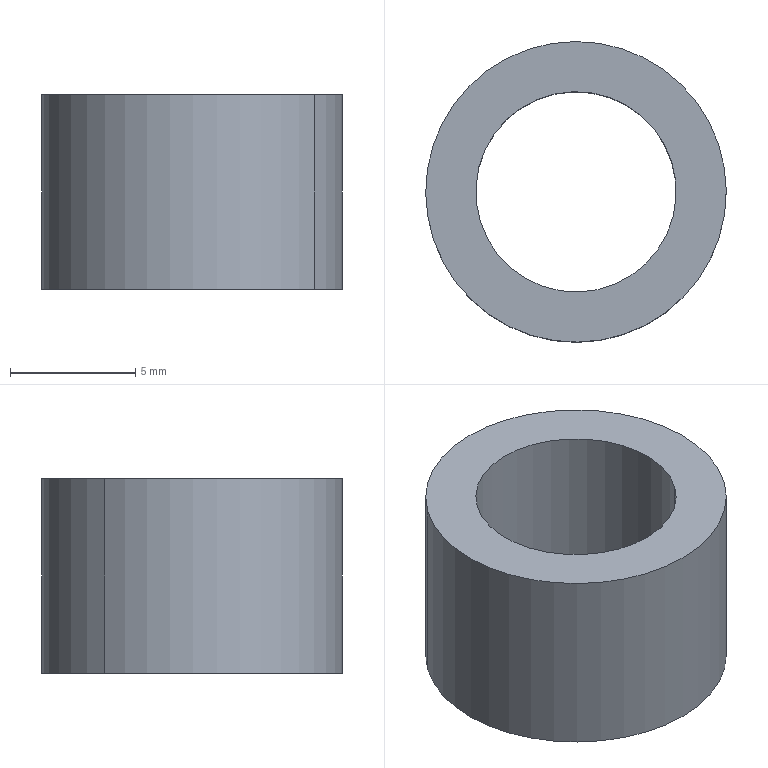Component | SolidWorks | 10BoltSleeve-Length7.75-2 | 1 solid | 6 faces | box 12 x 12 x 7.75 mm | volume 487 mm3 | cylinder 4 | plane 2 | commonest cylinder face diameters 8 x2 12 x2
build123d program:
from build123d import *

# Parameters (mm, degrees)
SKETCH1_R           = 6
SKETCH1_R_2         = 4
BOSS_EXTRUDE1_DEPTH = 7.75


with BuildPart() as part:
    # Sketch1 → Boss-Extrude1 (new body)
    with BuildSketch(Plane.XY):
        Circle(SKETCH1_R)
        Circle(SKETCH1_R_2, mode=Mode.SUBTRACT)
    extrude(amount=BOSS_EXTRUDE1_DEPTH)


solid = part.part

# Placed as in the assembly
solid = solid.moved(Location((94.618, 134.462, 31.788), (0, 0, 0)))
STEP:
#1=COLOUR_RGB('',0.7922,0.8196,0.9333);
#2=FILL_AREA_STYLE_COLOUR('',#1);
#3=FILL_AREA_STYLE('',(#2));
#4=SURFACE_STYLE_FILL_AREA(#3);
#5=SURFACE_SIDE_STYLE('',(#4));
#6=SURFACE_STYLE_USAGE(.BOTH.,#5);
#7=PRESENTATION_STYLE_ASSIGNMENT((#6));
#8=CARTESIAN_POINT('',(3.597,5.385,1.557));
#9=VERTEX_POINT('',#8);
#10=CARTESIAN_POINT('',(3.853,5.202,1.557));
#11=VERTEX_POINT('',#10);
#12=CARTESIAN_POINT('',(3.725,5.294,1.557));
#13=DIRECTION('',(0.,0.,1.));
#14=DIRECTION('',(0.8135,-0.5816,0.));
#15=AXIS2_PLACEMENT_3D('',#12,#13,#14);
#16=CIRCLE('',#15,0.1575);
#17=EDGE_CURVE('',#9,#11,#16,.T.);
#18=ORIENTED_EDGE('',*,*,#17,.T.);
#19=CARTESIAN_POINT('',(3.853,5.202,1.251));
#20=VERTEX_POINT('',#19);
#21=CARTESIAN_POINT('',(3.853,5.202,1.557));
#22=DIRECTION('',(0.,0.,-1.));
#23=VECTOR('',#22,39.37);
#24=LINE('',#21,#23);
#25=EDGE_CURVE('',#11,#20,#24,.T.);
#26=ORIENTED_EDGE('',*,*,#25,.T.);
#27=CARTESIAN_POINT('',(3.597,5.385,1.251));
#28=VERTEX_POINT('',#27);
#29=CARTESIAN_POINT('',(3.725,5.294,1.251));
#30=DIRECTION('',(0.,0.,1.));
#31=DIRECTION('',(0.8135,-0.5816,0.));
#32=AXIS2_PLACEMENT_3D('',#29,#30,#31);
#33=CIRCLE('',#32,0.1575);
#34=EDGE_CURVE('',#28,#20,#33,.T.);
#35=ORIENTED_EDGE('',*,*,#34,.F.);
#36=CARTESIAN_POINT('',(3.597,5.385,1.557));
#37=DIRECTION('',(0.,0.,-1.));
#38=VECTOR('',#37,39.37);
#39=LINE('',#36,#38);
#40=EDGE_CURVE('',#9,#28,#39,.T.);
#41=ORIENTED_EDGE('',*,*,#40,.F.);
#42=EDGE_LOOP('',(#18,#26,#35,#41));
#43=FACE_OUTER_BOUND('',#42,.T.);
#44=CARTESIAN_POINT('',(3.725,5.294,1.557));
#45=DIRECTION('',(0.,0.,-1.));
#46=DIRECTION('',(-0.8135,0.5816,0.));
#47=AXIS2_PLACEMENT_3D('',#44,#45,#46);
#48=CYLINDRICAL_SURFACE('',#47,0.1575);
#49=ADVANCED_FACE('',(#43),#48,.F.);
#50=CARTESIAN_POINT('',(3.917,5.156,1.557));
#51=VERTEX_POINT('',#50);
#52=CARTESIAN_POINT('',(3.533,5.431,1.557));
#53=VERTEX_POINT('',#52);
#54=CARTESIAN_POINT('',(3.725,5.294,1.557));
#55=DIRECTION('',(0.,0.,1.));
#56=DIRECTION('',(0.8135,-0.5816,0.));
#57=AXIS2_PLACEMENT_3D('',#54,#55,#56);
#58=CIRCLE('',#57,0.2362);
#59=EDGE_CURVE('',#51,#53,#58,.T.);
#60=ORIENTED_EDGE('',*,*,#59,.F.);
#61=CARTESIAN_POINT('',(3.917,5.156,1.251));
#62=VERTEX_POINT('',#61);
#63=CARTESIAN_POINT('',(3.917,5.156,1.557));
#64=DIRECTION('',(0.,0.,-1.));
#65=VECTOR('',#64,39.37);
#66=LINE('',#63,#65);
#67=EDGE_CURVE('',#51,#62,#66,.T.);
#68=ORIENTED_EDGE('',*,*,#67,.T.);
#69=CARTESIAN_POINT('',(3.533,5.431,1.251));
#70=VERTEX_POINT('',#69);
#71=CARTESIAN_POINT('',(3.725,5.294,1.251));
#72=DIRECTION('',(0.,0.,1.));
#73=DIRECTION('',(0.8135,-0.5816,0.));
#74=AXIS2_PLACEMENT_3D('',#71,#72,#73);
#75=CIRCLE('',#74,0.2362);
#76=EDGE_CURVE('',#62,#70,#75,.T.);
#77=ORIENTED_EDGE('',*,*,#76,.T.);
#78=CARTESIAN_POINT('',(3.533,5.431,1.557));
#79=DIRECTION('',(0.,0.,-1.));
#80=VECTOR('',#79,39.37);
#81=LINE('',#78,#80);
#82=EDGE_CURVE('',#53,#70,#81,.T.);
#83=ORIENTED_EDGE('',*,*,#82,.F.);
#84=EDGE_LOOP('',(#60,#68,#77,#83));
#85=FACE_OUTER_BOUND('',#84,.T.);
#86=CARTESIAN_POINT('',(3.725,5.294,1.557));
#87=DIRECTION('',(0.,0.,-1.));
#88=DIRECTION('',(-0.8135,0.5816,0.));
#89=AXIS2_PLACEMENT_3D('',#86,#87,#88);
#90=CYLINDRICAL_SURFACE('',#89,0.2362);
#91=ADVANCED_FACE('',(#85),#90,.T.);
#92=CARTESIAN_POINT('',(3.725,5.294,1.557));
#93=DIRECTION('',(0.,0.,1.));
#94=DIRECTION('',(0.8135,-0.5816,0.));
#95=AXIS2_PLACEMENT_3D('',#92,#93,#94);
#96=CIRCLE('',#95,0.2362);
#97=EDGE_CURVE('',#53,#51,#96,.T.);
#98=ORIENTED_EDGE('',*,*,#97,.T.);
#99=ORIENTED_EDGE('',*,*,#59,.T.);
#100=EDGE_LOOP('',(#98,#99));
#101=FACE_OUTER_BOUND('',#100,.T.);
#102=ORIENTED_EDGE('',*,*,#17,.F.);
#103=CARTESIAN_POINT('',(3.725,5.294,1.557));
#104=DIRECTION('',(0.,0.,1.));
#105=DIRECTION('',(0.8135,-0.5816,0.));
#106=AXIS2_PLACEMENT_3D('',#103,#104,#105);
#107=CIRCLE('',#106,0.1575);
#108=EDGE_CURVE('',#11,#9,#107,.T.);
#109=ORIENTED_EDGE('',*,*,#108,.F.);
#110=EDGE_LOOP('',(#102,#109));
#111=FACE_BOUND('',#110,.T.);
#112=CARTESIAN_POINT('',(3.725,5.294,1.557));
#113=DIRECTION('',(0.,0.,1.));
#114=DIRECTION('',(0.8135,-0.5816,0.));
#115=AXIS2_PLACEMENT_3D('',#112,#113,#114);
#116=PLANE('',#115);
#117=ADVANCED_FACE('',(#101,#111),#116,.T.);
#118=CARTESIAN_POINT('',(3.725,5.294,1.251));
#119=DIRECTION('',(0.,0.,1.));
#120=DIRECTION('',(0.8135,-0.5816,0.));
#121=AXIS2_PLACEMENT_3D('',#118,#119,#120);
#122=CIRCLE('',#121,0.2362);
#123=EDGE_CURVE('',#70,#62,#122,.T.);
#124=ORIENTED_EDGE('',*,*,#123,.F.);
#125=ORIENTED_EDGE('',*,*,#76,.F.);
#126=EDGE_LOOP('',(#124,#125));
#127=FACE_OUTER_BOUND('',#126,.T.);
#128=ORIENTED_EDGE('',*,*,#34,.T.);
#129=CARTESIAN_POINT('',(3.725,5.294,1.251));
#130=DIRECTION('',(0.,0.,1.));
#131=DIRECTION('',(0.8135,-0.5816,0.));
#132=AXIS2_PLACEMENT_3D('',#129,#130,#131);
#133=CIRCLE('',#132,0.1575);
#134=EDGE_CURVE('',#20,#28,#133,.T.);
#135=ORIENTED_EDGE('',*,*,#134,.T.);
#136=EDGE_LOOP('',(#128,#135));
#137=FACE_BOUND('',#136,.T.);
#138=CARTESIAN_POINT('',(3.725,5.294,1.251));
#139=DIRECTION('',(0.,0.,1.));
#140=DIRECTION('',(0.8135,-0.5816,0.));
#141=AXIS2_PLACEMENT_3D('',#138,#139,#140);
#142=PLANE('',#141);
#143=ADVANCED_FACE('',(#127,#137),#142,.F.);
#144=ORIENTED_EDGE('',*,*,#67,.F.);
#145=ORIENTED_EDGE('',*,*,#97,.F.);
#146=ORIENTED_EDGE('',*,*,#82,.T.);
#147=ORIENTED_EDGE('',*,*,#123,.T.);
#148=EDGE_LOOP('',(#144,#145,#146,#147));
#149=FACE_OUTER_BOUND('',#148,.T.);
#150=CARTESIAN_POINT('',(3.725,5.294,1.557));
#151=DIRECTION('',(0.,0.,-1.));
#152=DIRECTION('',(-0.8135,0.5816,0.));
#153=AXIS2_PLACEMENT_3D('',#150,#151,#152);
#154=CYLINDRICAL_SURFACE('',#153,0.2362);
#155=ADVANCED_FACE('',(#149),#154,.T.);
#156=ORIENTED_EDGE('',*,*,#25,.F.);
#157=ORIENTED_EDGE('',*,*,#108,.T.);
#158=ORIENTED_EDGE('',*,*,#40,.T.);
#159=ORIENTED_EDGE('',*,*,#134,.F.);
#160=EDGE_LOOP('',(#156,#157,#158,#159));
#161=FACE_OUTER_BOUND('',#160,.T.);
#162=CARTESIAN_POINT('',(3.725,5.294,1.557));
#163=DIRECTION('',(0.,0.,-1.));
#164=DIRECTION('',(-0.8135,0.5816,0.));
#165=AXIS2_PLACEMENT_3D('',#162,#163,#164);
#166=CYLINDRICAL_SURFACE('',#165,0.1575);
#167=ADVANCED_FACE('',(#161),#166,.F.);
#168=CLOSED_SHELL('',(#49,#91,#117,#143,#155,#167));
#169=MANIFOLD_SOLID_BREP('',#168);
#170=STYLED_ITEM('',(#7),#169);
#171=(LENGTH_UNIT()NAMED_UNIT(*)SI_UNIT($,.METRE.));
#172=LENGTH_MEASURE_WITH_UNIT(LENGTH_MEASURE(0.0254),#171);
#173=DIMENSIONAL_EXPONENTS(1.,0.,0.,0.,0.,0.,0.);
#174=(CONVERSION_BASED_UNIT('',#172)LENGTH_UNIT()NAMED_UNIT(#173));
#175=UNCERTAINTY_MEASURE_WITH_UNIT(LENGTH_MEASURE(0.00001),#174,'','');
#176=(NAMED_UNIT(*)PLANE_ANGLE_UNIT()SI_UNIT($,.RADIAN.));
#177=(NAMED_UNIT(*)SI_UNIT($,.STERADIAN.)SOLID_ANGLE_UNIT());
#178=(GEOMETRIC_REPRESENTATION_CONTEXT(3)GLOBAL_UNCERTAINTY_ASSIGNED_CONTEXT((#175))GLOBAL_UNIT_ASSIGNED_CONTEXT((#174,#176,#177))REPRESENTATION_CONTEXT('',''));
#179=MECHANICAL_DESIGN_GEOMETRIC_PRESENTATION_REPRESENTATION('',(#170),#178);
#180=CARTESIAN_POINT('',(0.,0.,0.));
#181=DIRECTION('',(0.,0.,1.));
#182=DIRECTION('',(1.,0.,0.));
#183=AXIS2_PLACEMENT_3D('',#180,#181,#182);
#184=(LENGTH_UNIT()NAMED_UNIT(*)SI_UNIT($,.METRE.));
#185=LENGTH_MEASURE_WITH_UNIT(LENGTH_MEASURE(0.0254),#184);
#186=DIMENSIONAL_EXPONENTS(1.,0.,0.,0.,0.,0.,0.);
#187=(CONVERSION_BASED_UNIT('',#185)LENGTH_UNIT()NAMED_UNIT(#186));
#188=UNCERTAINTY_MEASURE_WITH_UNIT(LENGTH_MEASURE(0.00001),#187,'','');
#189=(NAMED_UNIT(*)PLANE_ANGLE_UNIT()SI_UNIT($,.RADIAN.));
#190=(NAMED_UNIT(*)SI_UNIT($,.STERADIAN.)SOLID_ANGLE_UNIT());
#191=(GEOMETRIC_REPRESENTATION_CONTEXT(3)GLOBAL_UNCERTAINTY_ASSIGNED_CONTEXT((#188))GLOBAL_UNIT_ASSIGNED_CONTEXT((#187,#189,#190))REPRESENTATION_CONTEXT('',''));
#192=ADVANCED_BREP_SHAPE_REPRESENTATION('',(#169,#183),#191);
#193=PRESENTATION_LAYER_ASSIGNMENT('','',(#170));